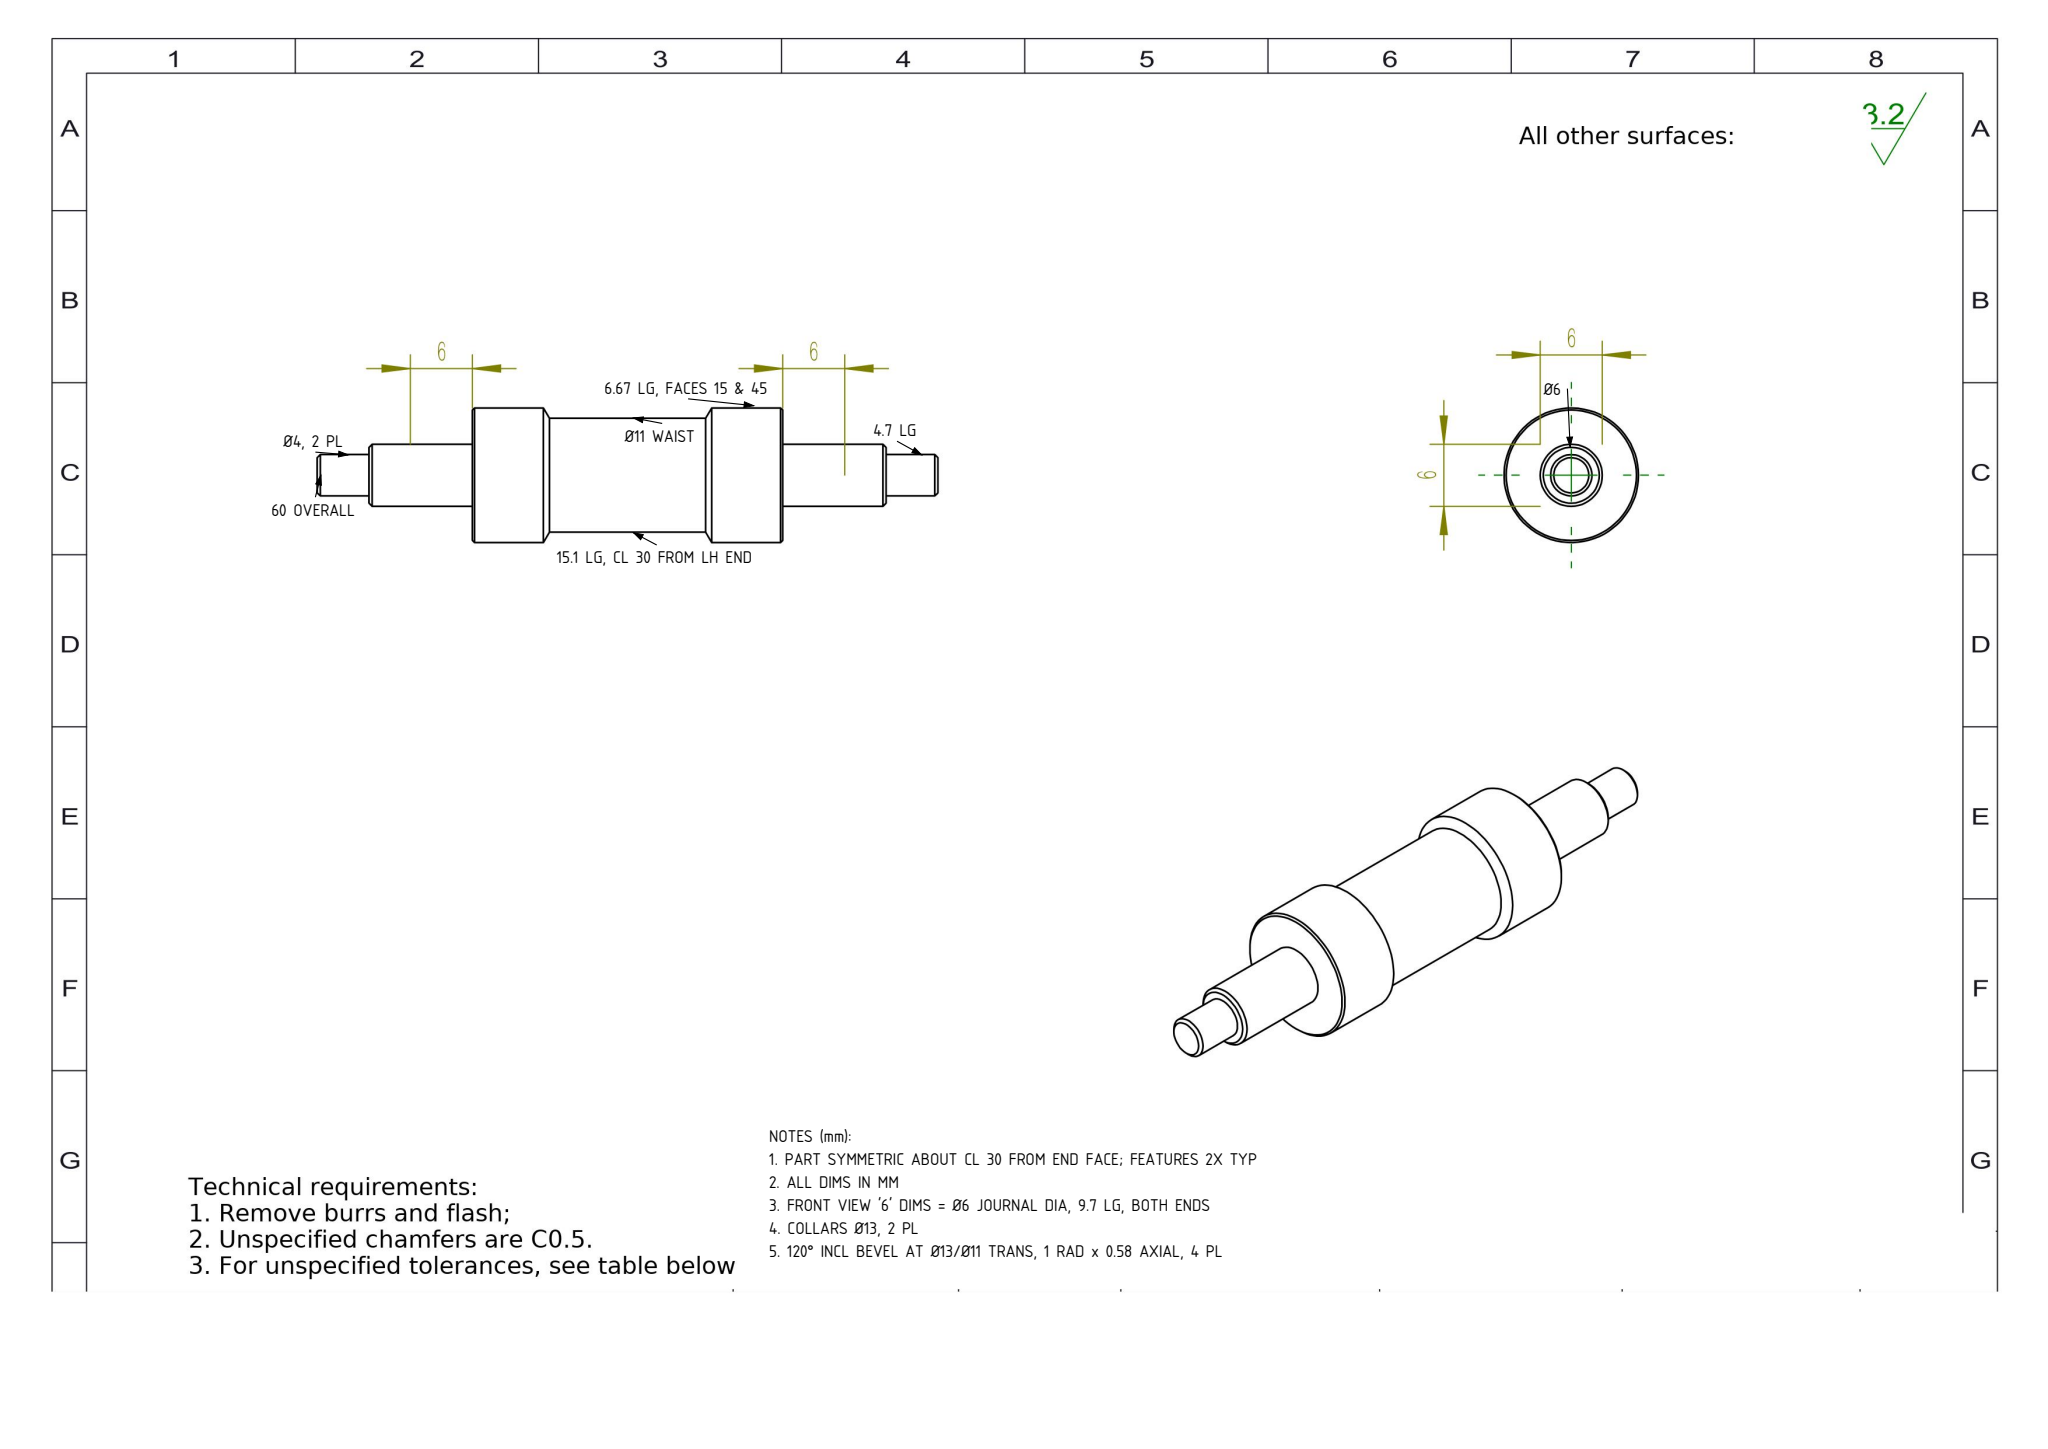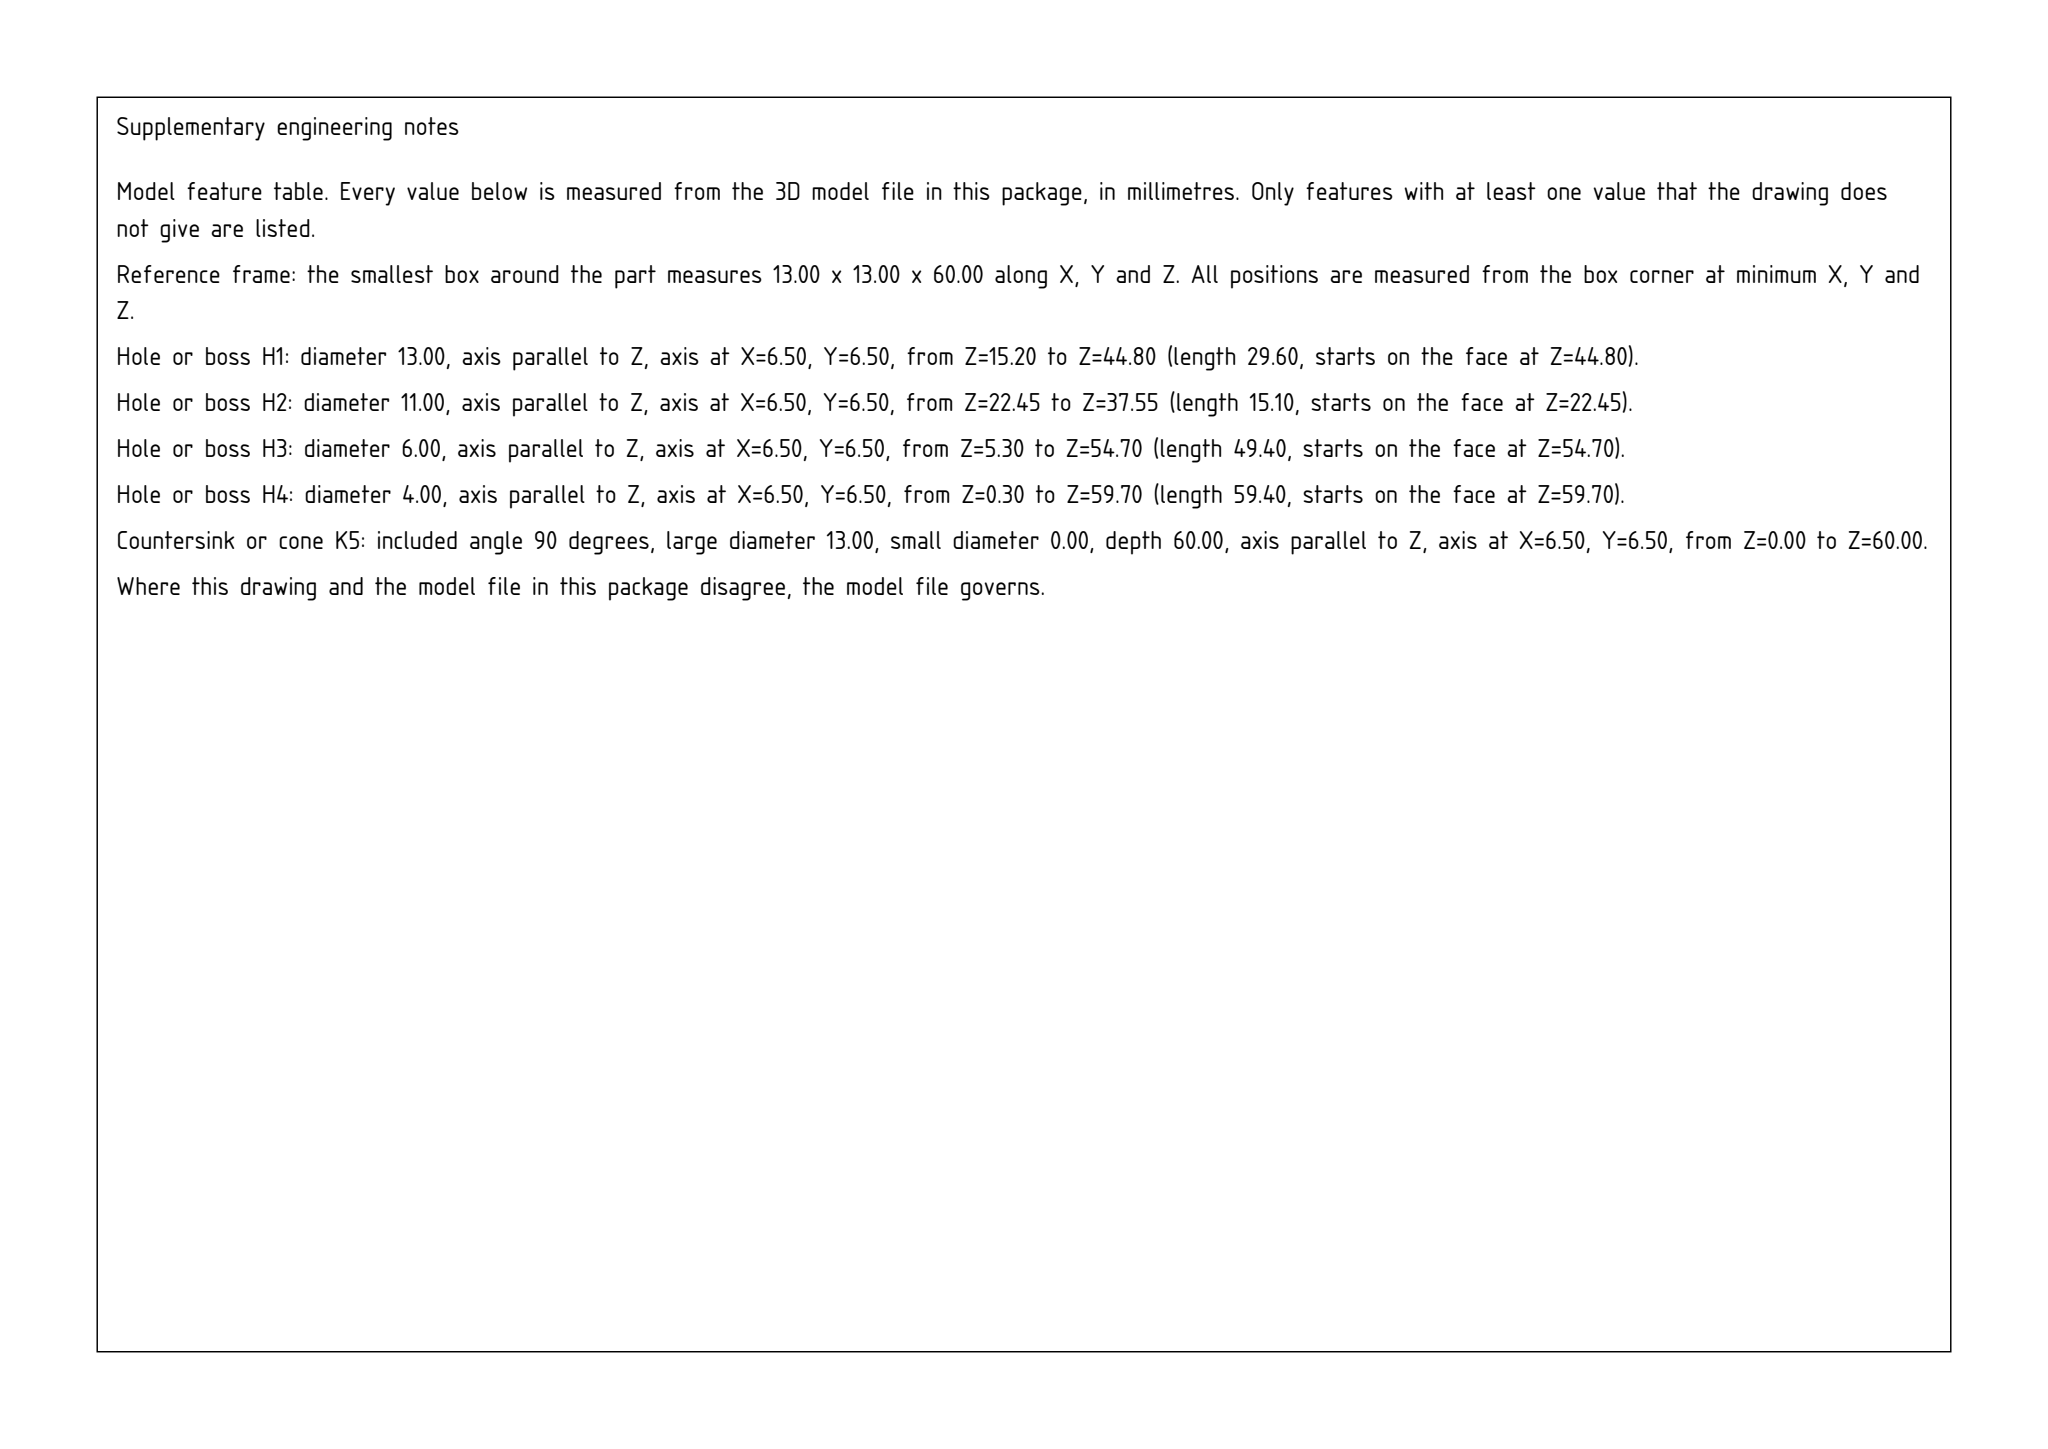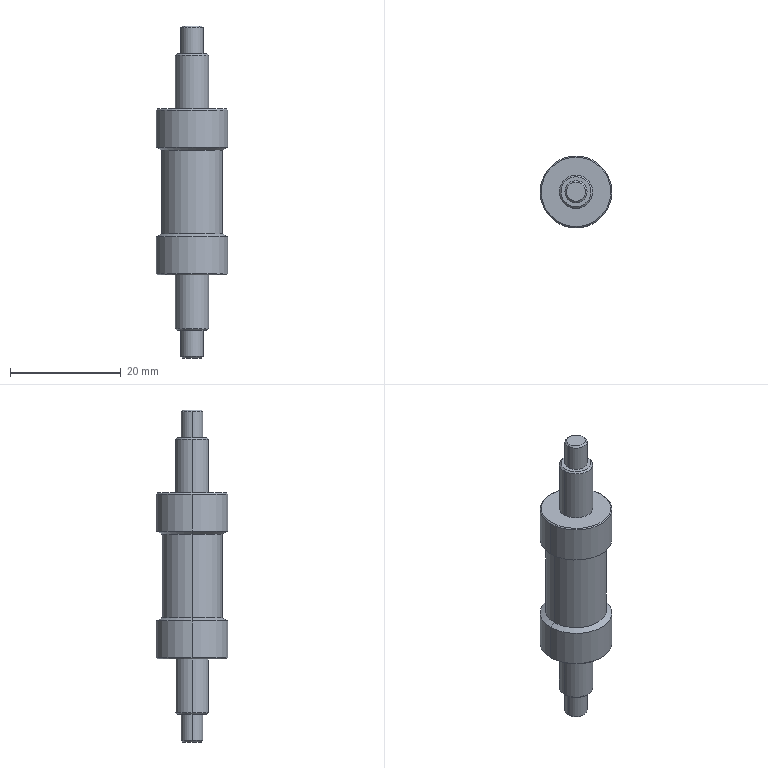Part | SolidWorks | mm | 1 solid | 36 faces | box 13 x 13 x 60 mm | volume 4077 mm3 | cone 16 | cylinder 14 | plane 6 | commonest cylinder face diameters 6 x4 4 x4 13 x4 11 x2
Drawing notes:
PART SYMMETRIC ABOUT CL 30 FROM END FACE; FEATURES 2X TYP | from the solid: mirrored plane set 0/60, 5/55, 15/45; cyl counts 2x per dia
ALL DIMS IN MM | from the solid: STEP model units mm; bbox 13.0 x 13.0 x 60.0
FRONT VIEW '6' DIMS = Ø6 JOURNAL DIA, 9.7 LG, BOTH ENDS | from the solid: cylinders: [6.0,'z',[6.5,6.5],9.7] x4 (stacked ends); end view shows 6 across both axes
COLLARS Ø13, 2 PL | from the solid: cylinders: dia 13.0 about z-axis at (6.5,6.5)
Ø13 COLLAR 6.67 LG; COLLAR FACES 15 & 45 FROM LH END FACE | from the solid: Ø13 length 6.67; axis planes z=5,15,45,55 on 60 long part
MIDDLE WAIST Ø11 | from the solid: cylinder dia 11.0 about z-axis
Ø11 WAIST 15.1 LG, CL AT 30 FROM LH END FACE | from the solid: Ø11 length 15.1; bbox z=60, symmetric about z=30
END STUBS Ø4, 2 PL | from the solid: cylinders dia 4.0 about z-axis, 4 faces
Ø4 STUB 4.7 LG EA END | from the solid: Ø4 cylinder length 4.7; z=0-4.7 and 55.3-60
OVERALL LG 60 END FACE TO END FACE | from the solid: bbox_xyz z = 60.0
120° INCL BEVEL AT Ø13/Ø11 TRANS, 1 RAD x 0.58 AXIAL, 4 PL | from the solid: cones 120.0 incl, ref dia 11.0 and 13.0, 2 ea
END VIEW: BOTH 6 DIMS = Ø6 INTERMEDIATE SHAFT DIA | from the solid: cylinder dia 6.0 about z-axis, concentric with Ø13 and Ø4
build123d program:
from build123d import *

# Parameters (mm, degrees)
SKETCH1_R               = 6.5
BOSS_EXTRUDE1_DEPTH     = 21
SKETCH5_R               = 2
BOSS_EXTRUDE2_DEPTH     = 30
SKETCH9_R               = 3
BOSS_EXTRUDE3_DEPTH     = 25
CHAMFER2_SIZE           = 0.3
SKETCH10_W              = 26
SKETCH10_H              = 26
SKETCH10_W_2            = 6
SKETCH10_H_2            = 6
CUT_EXTRUDE_THIN1_DEPTH = 6
SKETCH11_R              = 5
SKETCH11_R_2            = 3
CUT_EXTRUDE2_DEPTH      = 6
CHAMFER3_SIZE           = 0.2


with BuildPart() as part:
    # Sketch1 → Boss-Extrude1 (new, symmetric)
    with BuildSketch(Plane.XY):
        with Locations(Location((0, 0, 0), (0, 0, 180))):
            Circle(SKETCH1_R)
    extrude(amount=BOSS_EXTRUDE1_DEPTH, both=True)

    # Sketch5 → Boss-Extrude2 (add, symmetric)
    with BuildSketch(Plane.XY):
        Circle(SKETCH5_R)
    extrude(amount=BOSS_EXTRUDE2_DEPTH, both=True)

    # Sketch7 → Cut-Revolve2 (revolve, cut)
    with BuildSketch(Plane(origin=(0, 0, 0), x_dir=(0, 0, -1), z_dir=(1, 0, 0)), mode=Mode.PRIVATE) as cut_revolve2_sk:
        Polygon((-8.127, 6.5), (-7.55, 5.5), (7.55, 5.5), (8.127, 6.5), align=None)
    revolve(cut_revolve2_sk.sketch.rotate(Axis((0, 0, 30), (0, 0, -1)), 270), axis=Axis((0, 0, 30), (0, 0, -1)), mode=Mode.SUBTRACT)

    # Sketch9 → Boss-Extrude3 (add, symmetric)
    with BuildSketch(Plane.XY):
        Circle(SKETCH9_R)
    extrude(amount=BOSS_EXTRUDE3_DEPTH, both=True)

    # Chamfer2
    chamfer2_edges = [part.edges().sort_by_distance(p)[0] for p in [
        (6.5, 0, -21),
        (-3, 0, -25),
        (-3, 0, 25),
        (6.5, 0, 21),
        (-2, 0, -30),
        (-2, 0, 30),
    ]]
    chamfer(chamfer2_edges, length=CHAMFER2_SIZE)

    # Sketch10 → Cut-Extrude-Thin1 (cut)
    with BuildSketch(Plane.XY.offset(21)):
        Rectangle(SKETCH10_W, SKETCH10_H)
        Rectangle(SKETCH10_W_2, SKETCH10_H_2, mode=Mode.SUBTRACT)
    cut_extrude_thin1 = extrude(amount=-CUT_EXTRUDE_THIN1_DEPTH, mode=Mode.SUBTRACT)

    # Mirror1: Cut-Extrude-Thin1 across plane
    add(cut_extrude_thin1.mirror(Plane.XY), mode=Mode.SUBTRACT)

    # Sketch11 → Cut-Extrude2 (cut)
    with BuildSketch(Plane.XY.offset(21)):
        Circle(SKETCH11_R)
        Circle(SKETCH11_R_2, mode=Mode.SUBTRACT)
    cut_extrude2 = extrude(amount=-CUT_EXTRUDE2_DEPTH, mode=Mode.SUBTRACT)

    # Mirror3: Cut-Extrude2 across plane
    add(cut_extrude2.mirror(Plane.XY), mode=Mode.SUBTRACT)

    # Chamfer3
    chamfer3_edges = [part.edges().sort_by_distance(p)[0] for p in [
        (6.5, 0, 15),
        (6.5, 0, -15),
    ]]
    chamfer(chamfer3_edges, length=CHAMFER3_SIZE)


solid = part.part